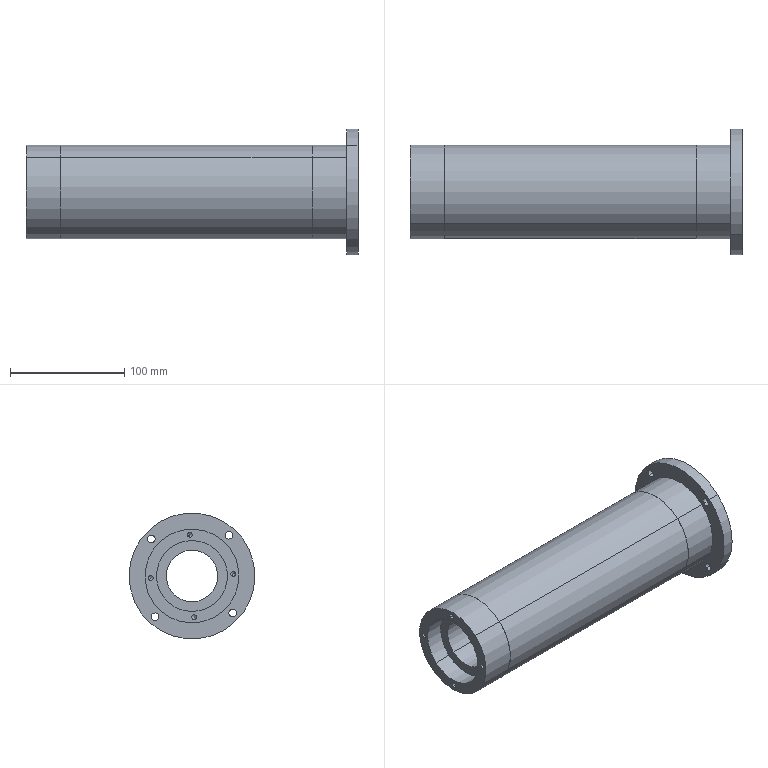Component | SolidWorks | 2-10-10WorkpieceAxisAssembly-1_2-10-1WorkpieceAxisBearingHousing-1 | 1 solid | 76 faces | volume 1049797 mm3 | cylinder 48 | cone 16 | plane 12 | commonest cylinder face diameters 4.2 x16 10 x8 6.6 x8 62 x4 82 x4 52 x2 45 x2 81.8 x2